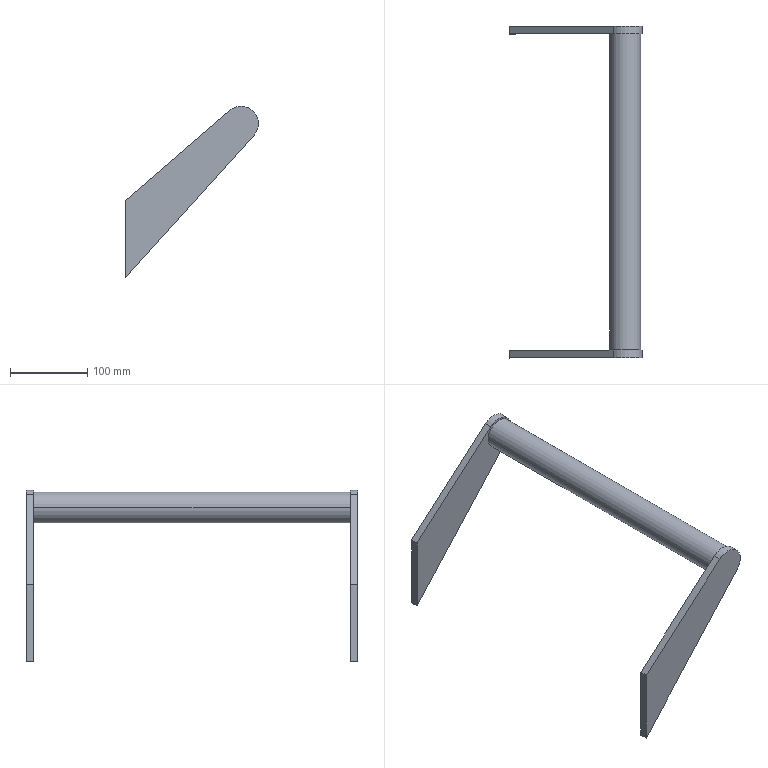Component | SolidWorks | Handle_2-2 | 1 solid | 18 faces | box 172.5 x 430 x 222.5 mm | volume 335928 mm3 | plane 12 | cylinder 6 | commonest cylinder face diameters 40 x2 45 x2 37 x2
STEP:
#1=COLOUR_RGB('',0.7922,0.8196,0.9333);
#2=FILL_AREA_STYLE_COLOUR('',#1);
#3=FILL_AREA_STYLE('',(#2));
#4=SURFACE_STYLE_FILL_AREA(#3);
#5=SURFACE_SIDE_STYLE('',(#4));
#6=SURFACE_STYLE_USAGE(.BOTH.,#5);
#7=PRESENTATION_STYLE_ASSIGNMENT((#6));
#8=CARTESIAN_POINT('',(26.375,9.434,79.254));
#9=VERTEX_POINT('',#8);
#10=CARTESIAN_POINT('',(27.95,9.434,79.254));
#11=VERTEX_POINT('',#10);
#12=CARTESIAN_POINT('',(27.163,9.434,79.254));
#13=DIRECTION('',(0.,1.,-0.));
#14=DIRECTION('',(-1.,0.,0.));
#15=AXIS2_PLACEMENT_3D('',#12,#13,#14);
#16=CIRCLE('',#15,0.7874);
#17=EDGE_CURVE('',#9,#11,#16,.T.);
#18=ORIENTED_EDGE('',*,*,#17,.F.);
#19=CARTESIAN_POINT('',(26.375,-6.708,79.254));
#20=VERTEX_POINT('',#19);
#21=CARTESIAN_POINT('',(26.375,9.828,79.254));
#22=DIRECTION('',(-0.,-1.,0.));
#23=VECTOR('',#22,39.37);
#24=LINE('',#21,#23);
#25=EDGE_CURVE('',#9,#20,#24,.T.);
#26=ORIENTED_EDGE('',*,*,#25,.T.);
#27=CARTESIAN_POINT('',(27.95,-6.708,79.254));
#28=VERTEX_POINT('',#27);
#29=CARTESIAN_POINT('',(27.163,-6.708,79.254));
#30=DIRECTION('',(-0.,-1.,0.));
#31=DIRECTION('',(-1.,0.,0.));
#32=AXIS2_PLACEMENT_3D('',#29,#30,#31);
#33=CIRCLE('',#32,0.7874);
#34=EDGE_CURVE('',#28,#20,#33,.T.);
#35=ORIENTED_EDGE('',*,*,#34,.F.);
#36=CARTESIAN_POINT('',(27.95,9.828,79.254));
#37=DIRECTION('',(-0.,-1.,0.));
#38=VECTOR('',#37,39.37);
#39=LINE('',#36,#38);
#40=EDGE_CURVE('',#11,#28,#39,.T.);
#41=ORIENTED_EDGE('',*,*,#40,.F.);
#42=EDGE_LOOP('',(#18,#26,#35,#41));
#43=FACE_OUTER_BOUND('',#42,.T.);
#44=CARTESIAN_POINT('',(27.163,9.828,79.254));
#45=DIRECTION('',(-0.,-1.,0.));
#46=DIRECTION('',(1.,0.,0.));
#47=AXIS2_PLACEMENT_3D('',#44,#45,#46);
#48=CYLINDRICAL_SURFACE('',#47,0.7874);
#49=ADVANCED_FACE('',(#43),#48,.T.);
#50=CARTESIAN_POINT('',(21.257,9.434,71.38));
#51=VERTEX_POINT('',#50);
#52=CARTESIAN_POINT('',(21.257,9.828,71.38));
#53=VERTEX_POINT('',#52);
#54=CARTESIAN_POINT('',(21.257,-7.101,71.38));
#55=DIRECTION('',(0.,1.,-0.));
#56=VECTOR('',#55,39.37);
#57=LINE('',#54,#56);
#58=EDGE_CURVE('',#51,#53,#57,.T.);
#59=ORIENTED_EDGE('',*,*,#58,.F.);
#60=CARTESIAN_POINT('',(21.257,9.434,75.317));
#61=VERTEX_POINT('',#60);
#62=CARTESIAN_POINT('',(21.257,9.434,71.38));
#63=DIRECTION('',(-0.,-0.,-1.));
#64=VECTOR('',#63,39.37);
#65=LINE('',#62,#64);
#66=EDGE_CURVE('',#61,#51,#65,.T.);
#67=ORIENTED_EDGE('',*,*,#66,.F.);
#68=CARTESIAN_POINT('',(21.257,9.828,75.317));
#69=VERTEX_POINT('',#68);
#70=CARTESIAN_POINT('',(21.257,-7.101,75.317));
#71=DIRECTION('',(0.,1.,-0.));
#72=VECTOR('',#71,39.37);
#73=LINE('',#70,#72);
#74=EDGE_CURVE('',#61,#69,#73,.T.);
#75=ORIENTED_EDGE('',*,*,#74,.T.);
#76=CARTESIAN_POINT('',(21.257,9.828,75.317));
#77=DIRECTION('',(-0.,-0.,-1.));
#78=VECTOR('',#77,39.37);
#79=LINE('',#76,#78);
#80=EDGE_CURVE('',#69,#53,#79,.T.);
#81=ORIENTED_EDGE('',*,*,#80,.T.);
#82=EDGE_LOOP('',(#59,#67,#75,#81));
#83=FACE_OUTER_BOUND('',#82,.T.);
#84=CARTESIAN_POINT('',(21.257,-7.101,75.317));
#85=DIRECTION('',(1.,-0.,-0.));
#86=DIRECTION('',(0.,0.,1.));
#87=AXIS2_PLACEMENT_3D('',#84,#85,#86);
#88=PLANE('',#87);
#89=ADVANCED_FACE('',(#83),#88,.F.);
#90=CARTESIAN_POINT('',(27.821,9.434,78.661));
#91=VERTEX_POINT('',#90);
#92=CARTESIAN_POINT('',(27.821,9.828,78.661));
#93=VERTEX_POINT('',#92);
#94=CARTESIAN_POINT('',(27.821,-7.101,78.661));
#95=DIRECTION('',(0.,1.,-0.));
#96=VECTOR('',#95,39.37);
#97=LINE('',#94,#96);
#98=EDGE_CURVE('',#91,#93,#97,.T.);
#99=ORIENTED_EDGE('',*,*,#98,.F.);
#100=CARTESIAN_POINT('',(21.257,9.434,71.38));
#101=DIRECTION('',(-0.6696,-0.,-0.7428));
#102=VECTOR('',#101,39.37);
#103=LINE('',#100,#102);
#104=EDGE_CURVE('',#91,#51,#103,.T.);
#105=ORIENTED_EDGE('',*,*,#104,.T.);
#106=ORIENTED_EDGE('',*,*,#58,.T.);
#107=CARTESIAN_POINT('',(21.257,9.828,71.38));
#108=DIRECTION('',(0.6696,0.,0.7428));
#109=VECTOR('',#108,39.37);
#110=LINE('',#107,#109);
#111=EDGE_CURVE('',#53,#93,#110,.T.);
#112=ORIENTED_EDGE('',*,*,#111,.T.);
#113=EDGE_LOOP('',(#99,#105,#106,#112));
#114=FACE_OUTER_BOUND('',#113,.T.);
#115=CARTESIAN_POINT('',(21.257,-7.101,71.38));
#116=DIRECTION('',(-0.7428,0.,0.6696));
#117=DIRECTION('',(-0.6696,-0.,-0.7428));
#118=AXIS2_PLACEMENT_3D('',#115,#116,#117);
#119=PLANE('',#118);
#120=ADVANCED_FACE('',(#114),#119,.F.);
#121=CARTESIAN_POINT('',(26.583,9.434,79.924));
#122=VERTEX_POINT('',#121);
#123=CARTESIAN_POINT('',(26.583,9.828,79.924));
#124=VERTEX_POINT('',#123);
#125=CARTESIAN_POINT('',(26.583,-7.101,79.924));
#126=DIRECTION('',(0.,1.,-0.));
#127=VECTOR('',#126,39.37);
#128=LINE('',#125,#127);
#129=EDGE_CURVE('',#122,#124,#128,.T.);
#130=ORIENTED_EDGE('',*,*,#129,.F.);
#131=CARTESIAN_POINT('',(27.163,9.434,79.254));
#132=DIRECTION('',(0.,1.,-0.));
#133=DIRECTION('',(-1.,0.,0.));
#134=AXIS2_PLACEMENT_3D('',#131,#132,#133);
#135=CIRCLE('',#134,0.8858);
#136=EDGE_CURVE('',#122,#91,#135,.T.);
#137=ORIENTED_EDGE('',*,*,#136,.T.);
#138=ORIENTED_EDGE('',*,*,#98,.T.);
#139=CARTESIAN_POINT('',(27.163,9.828,79.254));
#140=DIRECTION('',(-0.,-1.,0.));
#141=DIRECTION('',(1.,0.,0.));
#142=AXIS2_PLACEMENT_3D('',#139,#140,#141);
#143=CIRCLE('',#142,0.8858);
#144=EDGE_CURVE('',#93,#124,#143,.T.);
#145=ORIENTED_EDGE('',*,*,#144,.T.);
#146=EDGE_LOOP('',(#130,#137,#138,#145));
#147=FACE_OUTER_BOUND('',#146,.T.);
#148=CARTESIAN_POINT('',(27.163,-7.101,79.254));
#149=DIRECTION('',(0.,1.,-0.));
#150=DIRECTION('',(-1.,0.,0.));
#151=AXIS2_PLACEMENT_3D('',#148,#149,#150);
#152=CYLINDRICAL_SURFACE('',#151,0.8858);
#153=ADVANCED_FACE('',(#147),#152,.T.);
#154=ORIENTED_EDGE('',*,*,#74,.F.);
#155=CARTESIAN_POINT('',(26.583,9.434,79.924));
#156=DIRECTION('',(0.7563,0.,0.6542));
#157=VECTOR('',#156,39.37);
#158=LINE('',#155,#157);
#159=EDGE_CURVE('',#61,#122,#158,.T.);
#160=ORIENTED_EDGE('',*,*,#159,.T.);
#161=ORIENTED_EDGE('',*,*,#129,.T.);
#162=CARTESIAN_POINT('',(26.583,9.828,79.924));
#163=DIRECTION('',(-0.7563,-0.,-0.6542));
#164=VECTOR('',#163,39.37);
#165=LINE('',#162,#164);
#166=EDGE_CURVE('',#124,#69,#165,.T.);
#167=ORIENTED_EDGE('',*,*,#166,.T.);
#168=EDGE_LOOP('',(#154,#160,#161,#167));
#169=FACE_OUTER_BOUND('',#168,.T.);
#170=CARTESIAN_POINT('',(26.583,-7.101,79.924));
#171=DIRECTION('',(0.6542,-0.,-0.7563));
#172=DIRECTION('',(0.7563,0.,0.6542));
#173=AXIS2_PLACEMENT_3D('',#170,#171,#172);
#174=PLANE('',#173);
#175=ADVANCED_FACE('',(#169),#174,.F.);
#176=ORIENTED_EDGE('',*,*,#80,.F.);
#177=ORIENTED_EDGE('',*,*,#166,.F.);
#178=ORIENTED_EDGE('',*,*,#144,.F.);
#179=ORIENTED_EDGE('',*,*,#111,.F.);
#180=EDGE_LOOP('',(#176,#177,#178,#179));
#181=FACE_OUTER_BOUND('',#180,.T.);
#182=CARTESIAN_POINT('',(27.163,9.828,79.254));
#183=DIRECTION('',(-0.,-1.,0.));
#184=DIRECTION('',(1.,-0.,-0.));
#185=AXIS2_PLACEMENT_3D('',#182,#183,#184);
#186=PLANE('',#185);
#187=ADVANCED_FACE('',(#181),#186,.F.);
#188=CARTESIAN_POINT('',(27.163,9.434,79.254));
#189=DIRECTION('',(0.,1.,-0.));
#190=DIRECTION('',(-1.,0.,0.));
#191=AXIS2_PLACEMENT_3D('',#188,#189,#190);
#192=CIRCLE('',#191,0.7874);
#193=EDGE_CURVE('',#11,#9,#192,.T.);
#194=ORIENTED_EDGE('',*,*,#193,.T.);
#195=ORIENTED_EDGE('',*,*,#17,.T.);
#196=EDGE_LOOP('',(#194,#195));
#197=FACE_BOUND('',#196,.T.);
#198=ORIENTED_EDGE('',*,*,#136,.F.);
#199=ORIENTED_EDGE('',*,*,#159,.F.);
#200=ORIENTED_EDGE('',*,*,#66,.T.);
#201=ORIENTED_EDGE('',*,*,#104,.F.);
#202=EDGE_LOOP('',(#198,#199,#200,#201));
#203=FACE_OUTER_BOUND('',#202,.T.);
#204=CARTESIAN_POINT('',(21.257,9.434,71.38));
#205=DIRECTION('',(0.,1.,-0.));
#206=DIRECTION('',(-1.,0.,0.));
#207=AXIS2_PLACEMENT_3D('',#204,#205,#206);
#208=PLANE('',#207);
#209=ADVANCED_FACE('',(#197,#203),#208,.F.);
#210=ORIENTED_EDGE('',*,*,#25,.F.);
#211=ORIENTED_EDGE('',*,*,#193,.F.);
#212=ORIENTED_EDGE('',*,*,#40,.T.);
#213=CARTESIAN_POINT('',(27.163,-6.708,79.254));
#214=DIRECTION('',(-0.,-1.,0.));
#215=DIRECTION('',(-1.,0.,0.));
#216=AXIS2_PLACEMENT_3D('',#213,#214,#215);
#217=CIRCLE('',#216,0.7874);
#218=EDGE_CURVE('',#20,#28,#217,.T.);
#219=ORIENTED_EDGE('',*,*,#218,.F.);
#220=EDGE_LOOP('',(#210,#211,#212,#219));
#221=FACE_OUTER_BOUND('',#220,.T.);
#222=CARTESIAN_POINT('',(27.163,9.828,79.254));
#223=DIRECTION('',(-0.,-1.,0.));
#224=DIRECTION('',(1.,0.,0.));
#225=AXIS2_PLACEMENT_3D('',#222,#223,#224);
#226=CYLINDRICAL_SURFACE('',#225,0.7874);
#227=ADVANCED_FACE('',(#221),#226,.T.);
#228=CARTESIAN_POINT('',(21.257,-6.708,75.317));
#229=VERTEX_POINT('',#228);
#230=CARTESIAN_POINT('',(26.583,-6.708,79.924));
#231=VERTEX_POINT('',#230);
#232=CARTESIAN_POINT('',(26.583,-6.708,79.924));
#233=DIRECTION('',(0.7563,0.,0.6542));
#234=VECTOR('',#233,39.37);
#235=LINE('',#232,#234);
#236=EDGE_CURVE('',#229,#231,#235,.T.);
#237=ORIENTED_EDGE('',*,*,#236,.F.);
#238=CARTESIAN_POINT('',(21.257,-7.101,75.317));
#239=VERTEX_POINT('',#238);
#240=CARTESIAN_POINT('',(21.257,-7.101,75.317));
#241=DIRECTION('',(0.,1.,-0.));
#242=VECTOR('',#241,39.37);
#243=LINE('',#240,#242);
#244=EDGE_CURVE('',#239,#229,#243,.T.);
#245=ORIENTED_EDGE('',*,*,#244,.F.);
#246=CARTESIAN_POINT('',(26.583,-7.101,79.924));
#247=VERTEX_POINT('',#246);
#248=CARTESIAN_POINT('',(26.583,-7.101,79.924));
#249=DIRECTION('',(-0.7563,-0.,-0.6542));
#250=VECTOR('',#249,39.37);
#251=LINE('',#248,#250);
#252=EDGE_CURVE('',#247,#239,#251,.T.);
#253=ORIENTED_EDGE('',*,*,#252,.F.);
#254=CARTESIAN_POINT('',(26.583,-7.101,79.924));
#255=DIRECTION('',(0.,1.,-0.));
#256=VECTOR('',#255,39.37);
#257=LINE('',#254,#256);
#258=EDGE_CURVE('',#247,#231,#257,.T.);
#259=ORIENTED_EDGE('',*,*,#258,.T.);
#260=EDGE_LOOP('',(#237,#245,#253,#259));
#261=FACE_OUTER_BOUND('',#260,.T.);
#262=CARTESIAN_POINT('',(26.583,-7.101,79.924));
#263=DIRECTION('',(0.6542,-0.,-0.7563));
#264=DIRECTION('',(0.7563,0.,0.6542));
#265=AXIS2_PLACEMENT_3D('',#262,#263,#264);
#266=PLANE('',#265);
#267=ADVANCED_FACE('',(#261),#266,.F.);
#268=CARTESIAN_POINT('',(27.821,-6.708,78.661));
#269=VERTEX_POINT('',#268);
#270=CARTESIAN_POINT('',(27.163,-6.708,79.254));
#271=DIRECTION('',(0.,1.,-0.));
#272=DIRECTION('',(-1.,0.,0.));
#273=AXIS2_PLACEMENT_3D('',#270,#271,#272);
#274=CIRCLE('',#273,0.8858);
#275=EDGE_CURVE('',#231,#269,#274,.T.);
#276=ORIENTED_EDGE('',*,*,#275,.F.);
#277=ORIENTED_EDGE('',*,*,#258,.F.);
#278=CARTESIAN_POINT('',(27.821,-7.101,78.661));
#279=VERTEX_POINT('',#278);
#280=CARTESIAN_POINT('',(27.163,-7.101,79.254));
#281=DIRECTION('',(-0.,-1.,0.));
#282=DIRECTION('',(1.,0.,0.));
#283=AXIS2_PLACEMENT_3D('',#280,#281,#282);
#284=CIRCLE('',#283,0.8858);
#285=EDGE_CURVE('',#279,#247,#284,.T.);
#286=ORIENTED_EDGE('',*,*,#285,.F.);
#287=CARTESIAN_POINT('',(27.821,-7.101,78.661));
#288=DIRECTION('',(0.,1.,-0.));
#289=VECTOR('',#288,39.37);
#290=LINE('',#287,#289);
#291=EDGE_CURVE('',#279,#269,#290,.T.);
#292=ORIENTED_EDGE('',*,*,#291,.T.);
#293=EDGE_LOOP('',(#276,#277,#286,#292));
#294=FACE_OUTER_BOUND('',#293,.T.);
#295=CARTESIAN_POINT('',(27.163,-7.101,79.254));
#296=DIRECTION('',(0.,1.,-0.));
#297=DIRECTION('',(-1.,0.,0.));
#298=AXIS2_PLACEMENT_3D('',#295,#296,#297);
#299=CYLINDRICAL_SURFACE('',#298,0.8858);
#300=ADVANCED_FACE('',(#294),#299,.T.);
#301=CARTESIAN_POINT('',(21.257,-6.708,71.38));
#302=VERTEX_POINT('',#301);
#303=CARTESIAN_POINT('',(21.257,-6.708,71.38));
#304=DIRECTION('',(-0.6696,-0.,-0.7428));
#305=VECTOR('',#304,39.37);
#306=LINE('',#303,#305);
#307=EDGE_CURVE('',#269,#302,#306,.T.);
#308=ORIENTED_EDGE('',*,*,#307,.F.);
#309=ORIENTED_EDGE('',*,*,#291,.F.);
#310=CARTESIAN_POINT('',(21.257,-7.101,71.38));
#311=VERTEX_POINT('',#310);
#312=CARTESIAN_POINT('',(21.257,-7.101,71.38));
#313=DIRECTION('',(0.6696,0.,0.7428));
#314=VECTOR('',#313,39.37);
#315=LINE('',#312,#314);
#316=EDGE_CURVE('',#311,#279,#315,.T.);
#317=ORIENTED_EDGE('',*,*,#316,.F.);
#318=CARTESIAN_POINT('',(21.257,-7.101,71.38));
#319=DIRECTION('',(0.,1.,-0.));
#320=VECTOR('',#319,39.37);
#321=LINE('',#318,#320);
#322=EDGE_CURVE('',#311,#302,#321,.T.);
#323=ORIENTED_EDGE('',*,*,#322,.T.);
#324=EDGE_LOOP('',(#308,#309,#317,#323));
#325=FACE_OUTER_BOUND('',#324,.T.);
#326=CARTESIAN_POINT('',(21.257,-7.101,71.38));
#327=DIRECTION('',(-0.7428,0.,0.6696));
#328=DIRECTION('',(-0.6696,-0.,-0.7428));
#329=AXIS2_PLACEMENT_3D('',#326,#327,#328);
#330=PLANE('',#329);
#331=ADVANCED_FACE('',(#325),#330,.F.);
#332=CARTESIAN_POINT('',(21.257,-6.708,71.38));
#333=DIRECTION('',(-0.,-0.,-1.));
#334=VECTOR('',#333,39.37);
#335=LINE('',#332,#334);
#336=EDGE_CURVE('',#229,#302,#335,.T.);
#337=ORIENTED_EDGE('',*,*,#336,.T.);
#338=ORIENTED_EDGE('',*,*,#322,.F.);
#339=CARTESIAN_POINT('',(21.257,-7.101,75.317));
#340=DIRECTION('',(-0.,-0.,-1.));
#341=VECTOR('',#340,39.37);
#342=LINE('',#339,#341);
#343=EDGE_CURVE('',#239,#311,#342,.T.);
#344=ORIENTED_EDGE('',*,*,#343,.F.);
#345=ORIENTED_EDGE('',*,*,#244,.T.);
#346=EDGE_LOOP('',(#337,#338,#344,#345));
#347=FACE_OUTER_BOUND('',#346,.T.);
#348=CARTESIAN_POINT('',(21.257,-7.101,75.317));
#349=DIRECTION('',(1.,-0.,-0.));
#350=DIRECTION('',(0.,0.,1.));
#351=AXIS2_PLACEMENT_3D('',#348,#349,#350);
#352=PLANE('',#351);
#353=ADVANCED_FACE('',(#347),#352,.F.);
#354=ORIENTED_EDGE('',*,*,#34,.T.);
#355=ORIENTED_EDGE('',*,*,#218,.T.);
#356=EDGE_LOOP('',(#354,#355));
#357=FACE_BOUND('',#356,.T.);
#358=ORIENTED_EDGE('',*,*,#307,.T.);
#359=ORIENTED_EDGE('',*,*,#336,.F.);
#360=ORIENTED_EDGE('',*,*,#236,.T.);
#361=ORIENTED_EDGE('',*,*,#275,.T.);
#362=EDGE_LOOP('',(#358,#359,#360,#361));
#363=FACE_OUTER_BOUND('',#362,.T.);
#364=CARTESIAN_POINT('',(21.257,-6.708,71.38));
#365=DIRECTION('',(0.,1.,-0.));
#366=DIRECTION('',(-1.,0.,0.));
#367=AXIS2_PLACEMENT_3D('',#364,#365,#366);
#368=PLANE('',#367);
#369=ADVANCED_FACE('',(#357,#363),#368,.T.);
#370=ORIENTED_EDGE('',*,*,#343,.T.);
#371=ORIENTED_EDGE('',*,*,#316,.T.);
#372=ORIENTED_EDGE('',*,*,#285,.T.);
#373=ORIENTED_EDGE('',*,*,#252,.T.);
#374=EDGE_LOOP('',(#370,#371,#372,#373));
#375=FACE_OUTER_BOUND('',#374,.T.);
#376=CARTESIAN_POINT('',(27.163,-7.101,79.254));
#377=DIRECTION('',(-0.,-1.,0.));
#378=DIRECTION('',(1.,-0.,-0.));
#379=AXIS2_PLACEMENT_3D('',#376,#377,#378);
#380=PLANE('',#379);
#381=ADVANCED_FACE('',(#375),#380,.T.);
#382=CLOSED_SHELL('',(#49,#89,#120,#153,#175,#187,#209,#227,#267,#300,#331,#353,#369,#381));
#383=CARTESIAN_POINT('',(27.891,9.434,79.254));
#384=VERTEX_POINT('',#383);
#385=CARTESIAN_POINT('',(26.434,9.434,79.254));
#386=VERTEX_POINT('',#385);
#387=CARTESIAN_POINT('',(27.163,9.434,79.254));
#388=DIRECTION('',(0.,1.,-0.));
#389=DIRECTION('',(-1.,0.,0.));
#390=AXIS2_PLACEMENT_3D('',#387,#388,#389);
#391=CIRCLE('',#390,0.7283);
#392=EDGE_CURVE('',#384,#386,#391,.T.);
#393=ORIENTED_EDGE('',*,*,#392,.T.);
#394=CARTESIAN_POINT('',(26.434,-6.708,79.254));
#395=VERTEX_POINT('',#394);
#396=CARTESIAN_POINT('',(26.434,9.828,79.254));
#397=DIRECTION('',(-0.,-1.,0.));
#398=VECTOR('',#397,39.37);
#399=LINE('',#396,#398);
#400=EDGE_CURVE('',#386,#395,#399,.T.);
#401=ORIENTED_EDGE('',*,*,#400,.T.);
#402=CARTESIAN_POINT('',(27.891,-6.708,79.254));
#403=VERTEX_POINT('',#402);
#404=CARTESIAN_POINT('',(27.163,-6.708,79.254));
#405=DIRECTION('',(-0.,-1.,0.));
#406=DIRECTION('',(-1.,0.,0.));
#407=AXIS2_PLACEMENT_3D('',#404,#405,#406);
#408=CIRCLE('',#407,0.7283);
#409=EDGE_CURVE('',#395,#403,#408,.T.);
#410=ORIENTED_EDGE('',*,*,#409,.T.);
#411=CARTESIAN_POINT('',(27.891,9.828,79.254));
#412=DIRECTION('',(-0.,-1.,0.));
#413=VECTOR('',#412,39.37);
#414=LINE('',#411,#413);
#415=EDGE_CURVE('',#384,#403,#414,.T.);
#416=ORIENTED_EDGE('',*,*,#415,.F.);
#417=EDGE_LOOP('',(#393,#401,#410,#416));
#418=FACE_OUTER_BOUND('',#417,.T.);
#419=CARTESIAN_POINT('',(27.163,9.828,79.254));
#420=DIRECTION('',(-0.,-1.,0.));
#421=DIRECTION('',(1.,0.,0.));
#422=AXIS2_PLACEMENT_3D('',#419,#420,#421);
#423=CYLINDRICAL_SURFACE('',#422,0.7283);
#424=ADVANCED_FACE('',(#418),#423,.F.);
#425=ORIENTED_EDGE('',*,*,#392,.F.);
#426=CARTESIAN_POINT('',(27.163,9.434,79.254));
#427=DIRECTION('',(0.,1.,-0.));
#428=DIRECTION('',(-1.,0.,0.));
#429=AXIS2_PLACEMENT_3D('',#426,#427,#428);
#430=CIRCLE('',#429,0.7283);
#431=EDGE_CURVE('',#386,#384,#430,.T.);
#432=ORIENTED_EDGE('',*,*,#431,.F.);
#433=EDGE_LOOP('',(#425,#432));
#434=FACE_OUTER_BOUND('',#433,.T.);
#435=CARTESIAN_POINT('',(21.257,9.434,71.38));
#436=DIRECTION('',(0.,1.,-0.));
#437=DIRECTION('',(-1.,0.,0.));
#438=AXIS2_PLACEMENT_3D('',#435,#436,#437);
#439=PLANE('',#438);
#440=ADVANCED_FACE('',(#434),#439,.F.);
#441=ORIENTED_EDGE('',*,*,#400,.F.);
#442=ORIENTED_EDGE('',*,*,#431,.T.);
#443=ORIENTED_EDGE('',*,*,#415,.T.);
#444=CARTESIAN_POINT('',(27.163,-6.708,79.254));
#445=DIRECTION('',(-0.,-1.,0.));
#446=DIRECTION('',(-1.,0.,0.));
#447=AXIS2_PLACEMENT_3D('',#444,#445,#446);
#448=CIRCLE('',#447,0.7283);
#449=EDGE_CURVE('',#403,#395,#448,.T.);
#450=ORIENTED_EDGE('',*,*,#449,.T.);
#451=EDGE_LOOP('',(#441,#442,#443,#450));
#452=FACE_OUTER_BOUND('',#451,.T.);
#453=CARTESIAN_POINT('',(27.163,9.828,79.254));
#454=DIRECTION('',(-0.,-1.,0.));
#455=DIRECTION('',(1.,0.,0.));
#456=AXIS2_PLACEMENT_3D('',#453,#454,#455);
#457=CYLINDRICAL_SURFACE('',#456,0.7283);
#458=ADVANCED_FACE('',(#452),#457,.F.);
#459=ORIENTED_EDGE('',*,*,#449,.F.);
#460=ORIENTED_EDGE('',*,*,#409,.F.);
#461=EDGE_LOOP('',(#459,#460));
#462=FACE_OUTER_BOUND('',#461,.T.);
#463=CARTESIAN_POINT('',(21.257,-6.708,71.38));
#464=DIRECTION('',(0.,1.,-0.));
#465=DIRECTION('',(-1.,0.,0.));
#466=AXIS2_PLACEMENT_3D('',#463,#464,#465);
#467=PLANE('',#466);
#468=ADVANCED_FACE('',(#462),#467,.T.);
#469=CLOSED_SHELL('',(#424,#440,#458,#468));
#470=ORIENTED_CLOSED_SHELL('',*,#469,.F.);
#471=BREP_WITH_VOIDS('',#382,(#470));
#472=STYLED_ITEM('',(#7),#471);
#473=(LENGTH_UNIT()NAMED_UNIT(*)SI_UNIT($,.METRE.));
#474=LENGTH_MEASURE_WITH_UNIT(LENGTH_MEASURE(0.0254),#473);
#475=DIMENSIONAL_EXPONENTS(1.,0.,0.,0.,0.,0.,0.);
#476=(CONVERSION_BASED_UNIT('',#474)LENGTH_UNIT()NAMED_UNIT(#475));
#477=UNCERTAINTY_MEASURE_WITH_UNIT(LENGTH_MEASURE(0.00001),#476,'','');
#478=(NAMED_UNIT(*)PLANE_ANGLE_UNIT()SI_UNIT($,.RADIAN.));
#479=(NAMED_UNIT(*)SI_UNIT($,.STERADIAN.)SOLID_ANGLE_UNIT());
#480=(GEOMETRIC_REPRESENTATION_CONTEXT(3)GLOBAL_UNCERTAINTY_ASSIGNED_CONTEXT((#477))GLOBAL_UNIT_ASSIGNED_CONTEXT((#476,#478,#479))REPRESENTATION_CONTEXT('',''));
#481=MECHANICAL_DESIGN_GEOMETRIC_PRESENTATION_REPRESENTATION('',(#472),#480);
#482=CARTESIAN_POINT('',(0.,0.,0.));
#483=DIRECTION('',(0.,0.,1.));
#484=DIRECTION('',(1.,0.,0.));
#485=AXIS2_PLACEMENT_3D('',#482,#483,#484);
#486=(LENGTH_UNIT()NAMED_UNIT(*)SI_UNIT($,.METRE.));
#487=LENGTH_MEASURE_WITH_UNIT(LENGTH_MEASURE(0.0254),#486);
#488=DIMENSIONAL_EXPONENTS(1.,0.,0.,0.,0.,0.,0.);
#489=(CONVERSION_BASED_UNIT('',#487)LENGTH_UNIT()NAMED_UNIT(#488));
#490=UNCERTAINTY_MEASURE_WITH_UNIT(LENGTH_MEASURE(0.00001),#489,'','');
#491=(NAMED_UNIT(*)PLANE_ANGLE_UNIT()SI_UNIT($,.RADIAN.));
#492=(NAMED_UNIT(*)SI_UNIT($,.STERADIAN.)SOLID_ANGLE_UNIT());
#493=(GEOMETRIC_REPRESENTATION_CONTEXT(3)GLOBAL_UNCERTAINTY_ASSIGNED_CONTEXT((#490))GLOBAL_UNIT_ASSIGNED_CONTEXT((#489,#491,#492))REPRESENTATION_CONTEXT('',''));
#494=ADVANCED_BREP_SHAPE_REPRESENTATION('',(#471,#485),#493);
#495=PRESENTATION_LAYER_ASSIGNMENT('','',(#472));